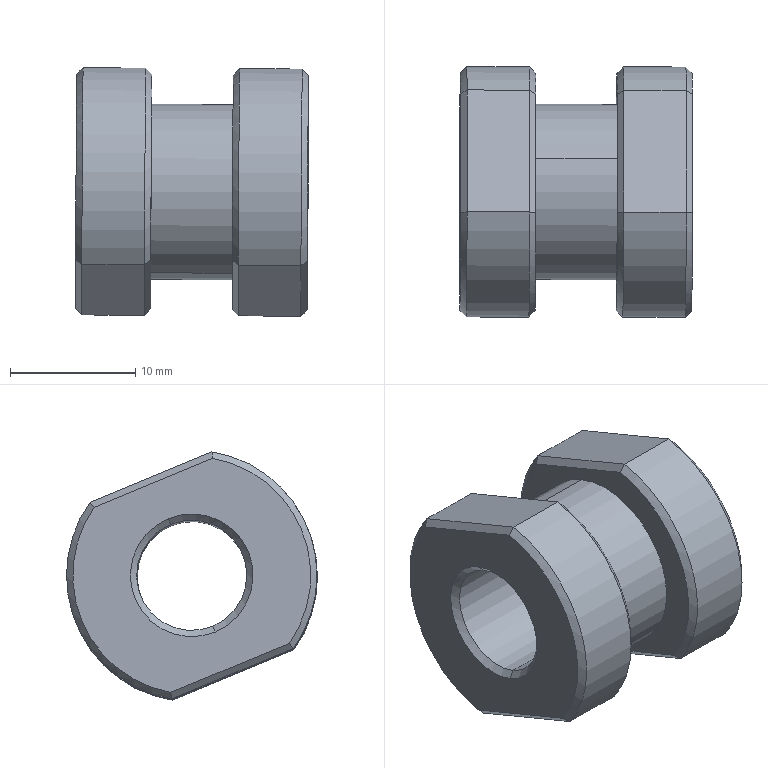Component | SolidWorks | CylinderConnector-1 | 1 solid | 36 faces | box 18.6 x 20.04 x 19.84 mm | volume 3351 mm3 | plane 16 | cone 12 | cylinder 8 | commonest cylinder face diameters 20 x4 8.8 x2 14 x2
build123d program:
from build123d import *

# Parameters (mm, degrees)
SKETCH1_R                   = 7
BOSS_EXTRUDE1_DEPTH         = 6.5
SKETCH2_R                   = 10
BOSS_EXTRUDE2_DEPTH         = 6
CUT_EXTRUDE1_DEPTH          = 24.286
M10X1_25_TAPPED_HOLE1_D     = 8.8
M10X1_25_TAPPED_HOLE1_DEPTH = 23.75
M10X1_25_TAPPED_HOLE1_TIP   = 2.644
CHAMFER1_SIZE               = 0.5


with BuildPart() as part:
    # Sketch1 → Boss-Extrude1 (new body)
    with BuildSketch(Plane.XY):
        with Locations(Location((0, 0, 0), (0, 0, 180))):
            Circle(SKETCH1_R)
    extrude(amount=BOSS_EXTRUDE1_DEPTH)

    # Sketch2 → Boss-Extrude2 (add)
    with BuildSketch(Plane.XY.offset(6.5)):
        Circle(SKETCH2_R)
    boss_extrude2 = extrude(amount=BOSS_EXTRUDE2_DEPTH)

    # Mirror1: Boss-Extrude2 across plane
    add(boss_extrude2.mirror(Plane(origin=(0, 0, 3.25), x_dir=(1, 0, 0), z_dir=(0, 0, -1))))

    # Sketch3 → Cut-Extrude1 (cut, through all)
    with BuildSketch(Plane.XY.offset(12.5)):
        with BuildLine():
            Line((8.5, 5.268), (8.5, -5.268))
            ThreePointArc((8.5, -5.268), (10, 0), (8.5, 5.268))
        make_face()
        with BuildLine():
            Line((-8.5, 5.268), (-8.5, -5.268))
            ThreePointArc((-8.5, -5.268), (-10, 0), (-8.5, 5.268))
        make_face()
    extrude(amount=-CUT_EXTRUDE1_DEPTH, mode=Mode.SUBTRACT)

    # M10x1.25 Tapped Hole1
    with Locations(Plane(origin=(0, 0, -6), x_dir=(-1, 0, 0), z_dir=(0, 0, -1))):
        with Locations((0, 0)):
            Hole(M10X1_25_TAPPED_HOLE1_D / 2, depth=M10X1_25_TAPPED_HOLE1_DEPTH)
            with Locations((0, 0, -(M10X1_25_TAPPED_HOLE1_DEPTH + M10X1_25_TAPPED_HOLE1_TIP / 2))):  # 118° drill point
                Cone(0, M10X1_25_TAPPED_HOLE1_D / 2, M10X1_25_TAPPED_HOLE1_TIP, mode=Mode.SUBTRACT)

    # Chamfer1
    chamfer1_edges = [part.edges().sort_by_distance(p)[0] for p in [
        (0, -10, -6),
        (0, -10, 0),
        (0, -10, 12.5),
        (0, -10, 6.5),
        (-8.5, 0, 6.5),
        (-8.5, 0, 0),
        (-8.5, 0, -6),
        (-8.5, 0, 12.5),
        (0, 10, -6),
        (0, 10, 0),
        (0, 10, 12.5),
        (0, 10, 6.5),
        (8.5, 0, 6.5),
        (8.5, 0, 0),
        (8.5, 0, -6),
        (8.5, 0, 12.5),
        (-4.4, 0, 12.5),
        (-4.4, 0, -6),
    ]]
    chamfer(chamfer1_edges, length=CHAMFER1_SIZE)


solid = part.part

# Placed as in the assembly
solid = solid.moved(Location((53.949, -72.168, 459.571), (158.758, 89.634, 178.758)))
STEP:
#1=CARTESIAN_POINT('',(2.595,-2.909,17.93));
#2=VERTEX_POINT('',#1);
#3=CARTESIAN_POINT('',(2.598,-2.776,18.251));
#4=VERTEX_POINT('',#3);
#5=CARTESIAN_POINT('',(2.596,-2.842,18.091));
#6=DIRECTION('',(1.,-0.002314,-0.005953));
#7=DIRECTION('',(0.006385,0.3824,0.924));
#8=AXIS2_PLACEMENT_3D('',#5,#6,#7);
#9=CIRCLE('',#8,0.1732);
#10=EDGE_CURVE('',#2,#4,#9,.T.);
#11=ORIENTED_EDGE('',*,*,#10,.F.);
#12=CARTESIAN_POINT('',(2.615,-2.916,17.912));
#13=VERTEX_POINT('',#12);
#14=CARTESIAN_POINT('',(2.595,-2.909,17.93));
#15=DIRECTION('',(0.7026,-0.272,-0.6576));
#16=VECTOR('',#15,39.37);
#17=LINE('',#14,#16);
#18=EDGE_CURVE('',#2,#13,#17,.T.);
#19=ORIENTED_EDGE('',*,*,#18,.T.);
#20=CARTESIAN_POINT('',(2.617,-2.769,18.269));
#21=VERTEX_POINT('',#20);
#22=CARTESIAN_POINT('',(2.616,-2.842,18.09));
#23=DIRECTION('',(-1.,0.002314,0.005953));
#24=DIRECTION('',(0.006385,0.3824,0.924));
#25=AXIS2_PLACEMENT_3D('',#22,#23,#24);
#26=CIRCLE('',#25,0.1929);
#27=EDGE_CURVE('',#21,#13,#26,.T.);
#28=ORIENTED_EDGE('',*,*,#27,.F.);
#29=CARTESIAN_POINT('',(2.598,-2.776,18.251));
#30=DIRECTION('',(0.7116,0.2688,0.6491));
#31=VECTOR('',#30,39.37);
#32=LINE('',#29,#31);
#33=EDGE_CURVE('',#4,#21,#32,.T.);
#34=ORIENTED_EDGE('',*,*,#33,.F.);
#35=EDGE_LOOP('',(#11,#19,#28,#34));
#36=FACE_OUTER_BOUND('',#35,.T.);
#37=CARTESIAN_POINT('',(2.596,-2.842,18.091));
#38=DIRECTION('',(1.,-0.002314,-0.005953));
#39=DIRECTION('',(0.006385,0.3824,0.924));
#40=AXIS2_PLACEMENT_3D('',#37,#38,#39);
#41=CONICAL_SURFACE('',#40,0.1732,0.7854);
#42=ADVANCED_FACE('',(#36),#41,.F.);
#43=CARTESIAN_POINT('',(1.909,-2.774,18.255));
#44=VERTEX_POINT('',#43);
#45=CARTESIAN_POINT('',(1.906,-2.907,17.935));
#46=VERTEX_POINT('',#45);
#47=CARTESIAN_POINT('',(1.907,-2.841,18.095));
#48=DIRECTION('',(-1.,0.002314,0.005953));
#49=DIRECTION('',(-0.006385,-0.3824,-0.924));
#50=AXIS2_PLACEMENT_3D('',#47,#48,#49);
#51=CIRCLE('',#50,0.1732);
#52=EDGE_CURVE('',#44,#46,#51,.T.);
#53=ORIENTED_EDGE('',*,*,#52,.F.);
#54=CARTESIAN_POINT('',(1.889,-2.767,18.273));
#55=VERTEX_POINT('',#54);
#56=CARTESIAN_POINT('',(1.909,-2.774,18.255));
#57=DIRECTION('',(-0.7026,0.272,0.6576));
#58=VECTOR('',#57,39.37);
#59=LINE('',#56,#58);
#60=EDGE_CURVE('',#44,#55,#59,.T.);
#61=ORIENTED_EDGE('',*,*,#60,.T.);
#62=CARTESIAN_POINT('',(1.887,-2.914,17.916));
#63=VERTEX_POINT('',#62);
#64=CARTESIAN_POINT('',(1.888,-2.841,18.095));
#65=DIRECTION('',(1.,-0.002314,-0.005953));
#66=DIRECTION('',(-0.006385,-0.3824,-0.924));
#67=AXIS2_PLACEMENT_3D('',#64,#65,#66);
#68=CIRCLE('',#67,0.1929);
#69=EDGE_CURVE('',#63,#55,#68,.T.);
#70=ORIENTED_EDGE('',*,*,#69,.F.);
#71=CARTESIAN_POINT('',(1.906,-2.907,17.935));
#72=DIRECTION('',(-0.7116,-0.2688,-0.6491));
#73=VECTOR('',#72,39.37);
#74=LINE('',#71,#73);
#75=EDGE_CURVE('',#46,#63,#74,.T.);
#76=ORIENTED_EDGE('',*,*,#75,.F.);
#77=EDGE_LOOP('',(#53,#61,#70,#76));
#78=FACE_OUTER_BOUND('',#77,.T.);
#79=CARTESIAN_POINT('',(1.907,-2.841,18.095));
#80=DIRECTION('',(-1.,0.002314,0.005953));
#81=DIRECTION('',(-0.006385,-0.3824,-0.924));
#82=AXIS2_PLACEMENT_3D('',#79,#80,#81);
#83=CONICAL_SURFACE('',#82,0.1732,0.7854);
#84=ADVANCED_FACE('',(#78),#83,.F.);
#85=ORIENTED_EDGE('',*,*,#10,.T.);
#86=CARTESIAN_POINT('',(1.889,-2.774,18.255));
#87=DIRECTION('',(-1.,0.002314,0.005953));
#88=VECTOR('',#87,39.37);
#89=LINE('',#86,#88);
#90=EDGE_CURVE('',#4,#44,#89,.T.);
#91=ORIENTED_EDGE('',*,*,#90,.T.);
#92=ORIENTED_EDGE('',*,*,#52,.T.);
#93=CARTESIAN_POINT('',(1.887,-2.907,17.935));
#94=DIRECTION('',(-1.,0.002314,0.005953));
#95=VECTOR('',#94,39.37);
#96=LINE('',#93,#95);
#97=EDGE_CURVE('',#2,#46,#96,.T.);
#98=ORIENTED_EDGE('',*,*,#97,.F.);
#99=EDGE_LOOP('',(#85,#91,#92,#98));
#100=FACE_OUTER_BOUND('',#99,.T.);
#101=CARTESIAN_POINT('',(1.888,-2.841,18.095));
#102=DIRECTION('',(-1.,0.002314,0.005953));
#103=DIRECTION('',(-0.006385,-0.3824,-0.924));
#104=AXIS2_PLACEMENT_3D('',#101,#102,#103);
#105=CYLINDRICAL_SURFACE('',#104,0.1732);
#106=ADVANCED_FACE('',(#100),#105,.F.);
#107=CARTESIAN_POINT('',(2.382,-2.736,18.346));
#108=VERTEX_POINT('',#107);
#109=CARTESIAN_POINT('',(2.378,-2.947,17.837));
#110=VERTEX_POINT('',#109);
#111=CARTESIAN_POINT('',(2.38,-2.842,18.092));
#112=DIRECTION('',(1.,-0.002314,-0.005953));
#113=DIRECTION('',(0.006385,0.3824,0.924));
#114=AXIS2_PLACEMENT_3D('',#111,#112,#113);
#115=CIRCLE('',#114,0.2756);
#116=EDGE_CURVE('',#108,#110,#115,.T.);
#117=ORIENTED_EDGE('',*,*,#116,.F.);
#118=CARTESIAN_POINT('',(2.126,-2.736,18.348));
#119=VERTEX_POINT('',#118);
#120=CARTESIAN_POINT('',(2.382,-2.736,18.346));
#121=DIRECTION('',(-1.,0.002314,0.005953));
#122=VECTOR('',#121,39.37);
#123=LINE('',#120,#122);
#124=EDGE_CURVE('',#108,#119,#123,.T.);
#125=ORIENTED_EDGE('',*,*,#124,.T.);
#126=CARTESIAN_POINT('',(2.122,-2.947,17.839));
#127=VERTEX_POINT('',#126);
#128=CARTESIAN_POINT('',(2.124,-2.841,18.093));
#129=DIRECTION('',(-1.,0.002314,0.005953));
#130=DIRECTION('',(-0.006385,-0.3824,-0.924));
#131=AXIS2_PLACEMENT_3D('',#128,#129,#130);
#132=CIRCLE('',#131,0.2756);
#133=EDGE_CURVE('',#127,#119,#132,.T.);
#134=ORIENTED_EDGE('',*,*,#133,.F.);
#135=CARTESIAN_POINT('',(2.378,-2.947,17.837));
#136=DIRECTION('',(-1.,0.002314,0.005953));
#137=VECTOR('',#136,39.37);
#138=LINE('',#135,#137);
#139=EDGE_CURVE('',#110,#127,#138,.T.);
#140=ORIENTED_EDGE('',*,*,#139,.F.);
#141=EDGE_LOOP('',(#117,#125,#134,#140));
#142=FACE_OUTER_BOUND('',#141,.T.);
#143=CARTESIAN_POINT('',(2.38,-2.842,18.092));
#144=DIRECTION('',(-1.,0.002314,0.005953));
#145=DIRECTION('',(-0.006385,-0.3824,-0.924));
#146=AXIS2_PLACEMENT_3D('',#143,#144,#145);
#147=CYLINDRICAL_SURFACE('',#146,0.2756);
#148=ADVANCED_FACE('',(#142),#147,.T.);
#149=CARTESIAN_POINT('',(2.397,-3.161,17.862));
#150=VERTEX_POINT('',#149);
#151=CARTESIAN_POINT('',(2.594,-3.162,17.861));
#152=VERTEX_POINT('',#151);
#153=CARTESIAN_POINT('',(1.886,-3.16,17.865));
#154=DIRECTION('',(1.,-0.002314,-0.005953));
#155=VECTOR('',#154,39.37);
#156=LINE('',#153,#155);
#157=EDGE_CURVE('',#150,#152,#156,.T.);
#158=ORIENTED_EDGE('',*,*,#157,.T.);
#159=CARTESIAN_POINT('',(2.599,-2.906,18.479));
#160=VERTEX_POINT('',#159);
#161=CARTESIAN_POINT('',(2.596,-2.842,18.091));
#162=DIRECTION('',(-1.,0.002314,0.005953));
#163=DIRECTION('',(0.006385,0.3824,0.924));
#164=AXIS2_PLACEMENT_3D('',#161,#162,#163);
#165=CIRCLE('',#164,0.3937);
#166=EDGE_CURVE('',#152,#160,#165,.T.);
#167=ORIENTED_EDGE('',*,*,#166,.T.);
#168=CARTESIAN_POINT('',(2.402,-2.906,18.48));
#169=VERTEX_POINT('',#168);
#170=CARTESIAN_POINT('',(1.89,-2.904,18.483));
#171=DIRECTION('',(1.,-0.002314,-0.005953));
#172=VECTOR('',#171,39.37);
#173=LINE('',#170,#172);
#174=EDGE_CURVE('',#169,#160,#173,.T.);
#175=ORIENTED_EDGE('',*,*,#174,.F.);
#176=CARTESIAN_POINT('',(2.4,-2.842,18.092));
#177=DIRECTION('',(1.,-0.002314,-0.005953));
#178=DIRECTION('',(0.006385,0.3824,0.924));
#179=AXIS2_PLACEMENT_3D('',#176,#177,#178);
#180=CIRCLE('',#179,0.3937);
#181=EDGE_CURVE('',#169,#150,#180,.T.);
#182=ORIENTED_EDGE('',*,*,#181,.T.);
#183=EDGE_LOOP('',(#158,#167,#175,#182));
#184=FACE_OUTER_BOUND('',#183,.T.);
#185=CARTESIAN_POINT('',(2.616,-2.842,18.09));
#186=DIRECTION('',(-1.,0.002314,0.005953));
#187=DIRECTION('',(-0.006385,-0.3824,-0.924));
#188=AXIS2_PLACEMENT_3D('',#185,#186,#187);
#189=CYLINDRICAL_SURFACE('',#188,0.3937);
#190=ADVANCED_FACE('',(#184),#189,.T.);
#191=CARTESIAN_POINT('',(1.905,-2.777,17.706));
#192=VERTEX_POINT('',#191);
#193=CARTESIAN_POINT('',(2.102,-2.778,17.705));
#194=VERTEX_POINT('',#193);
#195=CARTESIAN_POINT('',(1.886,-2.777,17.706));
#196=DIRECTION('',(1.,-0.002314,-0.005953));
#197=VECTOR('',#196,39.37);
#198=LINE('',#195,#197);
#199=EDGE_CURVE('',#192,#194,#198,.T.);
#200=ORIENTED_EDGE('',*,*,#199,.F.);
#201=CARTESIAN_POINT('',(1.91,-2.521,18.325));
#202=VERTEX_POINT('',#201);
#203=CARTESIAN_POINT('',(1.907,-2.841,18.095));
#204=DIRECTION('',(1.,-0.002314,-0.005953));
#205=DIRECTION('',(-0.006385,-0.3824,-0.924));
#206=AXIS2_PLACEMENT_3D('',#203,#204,#205);
#207=CIRCLE('',#206,0.3937);
#208=EDGE_CURVE('',#192,#202,#207,.T.);
#209=ORIENTED_EDGE('',*,*,#208,.T.);
#210=CARTESIAN_POINT('',(2.106,-2.522,18.323));
#211=VERTEX_POINT('',#210);
#212=CARTESIAN_POINT('',(1.89,-2.521,18.325));
#213=DIRECTION('',(1.,-0.002314,-0.005953));
#214=VECTOR('',#213,39.37);
#215=LINE('',#212,#214);
#216=EDGE_CURVE('',#202,#211,#215,.T.);
#217=ORIENTED_EDGE('',*,*,#216,.T.);
#218=CARTESIAN_POINT('',(2.104,-2.841,18.093));
#219=DIRECTION('',(-1.,0.002314,0.005953));
#220=DIRECTION('',(-0.006385,-0.3824,-0.924));
#221=AXIS2_PLACEMENT_3D('',#218,#219,#220);
#222=CIRCLE('',#221,0.3937);
#223=EDGE_CURVE('',#211,#194,#222,.T.);
#224=ORIENTED_EDGE('',*,*,#223,.T.);
#225=EDGE_LOOP('',(#200,#209,#217,#224));
#226=FACE_OUTER_BOUND('',#225,.T.);
#227=CARTESIAN_POINT('',(1.888,-2.841,18.095));
#228=DIRECTION('',(1.,-0.002314,-0.005953));
#229=DIRECTION('',(0.006385,0.3824,0.924));
#230=AXIS2_PLACEMENT_3D('',#227,#228,#229);
#231=CYLINDRICAL_SURFACE('',#230,0.3937);
#232=ADVANCED_FACE('',(#226),#231,.T.);
#233=ORIENTED_EDGE('',*,*,#124,.F.);
#234=CARTESIAN_POINT('',(2.38,-2.842,18.092));
#235=DIRECTION('',(1.,-0.002314,-0.005953));
#236=DIRECTION('',(0.006385,0.3824,0.924));
#237=AXIS2_PLACEMENT_3D('',#234,#235,#236);
#238=CIRCLE('',#237,0.2756);
#239=EDGE_CURVE('',#110,#108,#238,.T.);
#240=ORIENTED_EDGE('',*,*,#239,.F.);
#241=ORIENTED_EDGE('',*,*,#139,.T.);
#242=CARTESIAN_POINT('',(2.124,-2.841,18.093));
#243=DIRECTION('',(-1.,0.002314,0.005953));
#244=DIRECTION('',(-0.006385,-0.3824,-0.924));
#245=AXIS2_PLACEMENT_3D('',#242,#243,#244);
#246=CIRCLE('',#245,0.2756);
#247=EDGE_CURVE('',#119,#127,#246,.T.);
#248=ORIENTED_EDGE('',*,*,#247,.F.);
#249=EDGE_LOOP('',(#233,#240,#241,#248));
#250=FACE_OUTER_BOUND('',#249,.T.);
#251=CARTESIAN_POINT('',(2.38,-2.842,18.092));
#252=DIRECTION('',(-1.,0.002314,0.005953));
#253=DIRECTION('',(-0.006385,-0.3824,-0.924));
#254=AXIS2_PLACEMENT_3D('',#251,#252,#253);
#255=CYLINDRICAL_SURFACE('',#254,0.2756);
#256=ADVANCED_FACE('',(#250),#255,.T.);
#257=CARTESIAN_POINT('',(2.382,-2.535,18.306));
#258=VERTEX_POINT('',#257);
#259=CARTESIAN_POINT('',(2.378,-2.776,17.724));
#260=VERTEX_POINT('',#259);
#261=CARTESIAN_POINT('',(2.38,-2.842,18.092));
#262=DIRECTION('',(-1.,0.002314,0.005953));
#263=DIRECTION('',(0.006385,0.3824,0.924));
#264=AXIS2_PLACEMENT_3D('',#261,#262,#263);
#265=CIRCLE('',#264,0.374);
#266=EDGE_CURVE('',#258,#260,#265,.T.);
#267=ORIENTED_EDGE('',*,*,#266,.T.);
#268=CARTESIAN_POINT('',(2.378,-3.149,17.878));
#269=VERTEX_POINT('',#268);
#270=CARTESIAN_POINT('',(2.378,-2.962,17.801));
#271=DIRECTION('',(0.0001384,-0.924,0.3824));
#272=VECTOR('',#271,39.37);
#273=LINE('',#270,#272);
#274=EDGE_CURVE('',#260,#269,#273,.T.);
#275=ORIENTED_EDGE('',*,*,#274,.T.);
#276=CARTESIAN_POINT('',(2.382,-2.908,18.46));
#277=VERTEX_POINT('',#276);
#278=CARTESIAN_POINT('',(2.38,-2.842,18.092));
#279=DIRECTION('',(-1.,0.002314,0.005953));
#280=DIRECTION('',(0.006385,0.3824,0.924));
#281=AXIS2_PLACEMENT_3D('',#278,#279,#280);
#282=CIRCLE('',#281,0.374);
#283=EDGE_CURVE('',#269,#277,#282,.T.);
#284=ORIENTED_EDGE('',*,*,#283,.T.);
#285=CARTESIAN_POINT('',(2.382,-2.721,18.383));
#286=DIRECTION('',(-0.0001384,0.924,-0.3824));
#287=VECTOR('',#286,39.37);
#288=LINE('',#285,#287);
#289=EDGE_CURVE('',#277,#258,#288,.T.);
#290=ORIENTED_EDGE('',*,*,#289,.T.);
#291=EDGE_LOOP('',(#267,#275,#284,#290));
#292=FACE_OUTER_BOUND('',#291,.T.);
#293=ORIENTED_EDGE('',*,*,#239,.T.);
#294=ORIENTED_EDGE('',*,*,#116,.T.);
#295=EDGE_LOOP('',(#293,#294));
#296=FACE_BOUND('',#295,.T.);
#297=CARTESIAN_POINT('',(2.38,-2.842,18.092));
#298=DIRECTION('',(1.,-0.002314,-0.005953));
#299=DIRECTION('',(0.006385,0.3824,0.924));
#300=AXIS2_PLACEMENT_3D('',#297,#298,#299);
#301=PLANE('',#300);
#302=ADVANCED_FACE('',(#292,#296),#301,.F.);
#303=CARTESIAN_POINT('',(2.402,-2.522,18.322));
#304=VERTEX_POINT('',#303);
#305=CARTESIAN_POINT('',(2.599,-2.523,18.32));
#306=VERTEX_POINT('',#305);
#307=CARTESIAN_POINT('',(1.89,-2.521,18.325));
#308=DIRECTION('',(1.,-0.002314,-0.005953));
#309=VECTOR('',#308,39.37);
#310=LINE('',#307,#309);
#311=EDGE_CURVE('',#304,#306,#310,.T.);
#312=ORIENTED_EDGE('',*,*,#311,.T.);
#313=CARTESIAN_POINT('',(2.594,-2.779,17.702));
#314=VERTEX_POINT('',#313);
#315=CARTESIAN_POINT('',(2.596,-2.842,18.091));
#316=DIRECTION('',(-1.,0.002314,0.005953));
#317=DIRECTION('',(0.006385,0.3824,0.924));
#318=AXIS2_PLACEMENT_3D('',#315,#316,#317);
#319=CIRCLE('',#318,0.3937);
#320=EDGE_CURVE('',#306,#314,#319,.T.);
#321=ORIENTED_EDGE('',*,*,#320,.T.);
#322=CARTESIAN_POINT('',(2.397,-2.778,17.703));
#323=VERTEX_POINT('',#322);
#324=CARTESIAN_POINT('',(1.886,-2.777,17.706));
#325=DIRECTION('',(1.,-0.002314,-0.005953));
#326=VECTOR('',#325,39.37);
#327=LINE('',#324,#326);
#328=EDGE_CURVE('',#323,#314,#327,.T.);
#329=ORIENTED_EDGE('',*,*,#328,.F.);
#330=CARTESIAN_POINT('',(2.4,-2.842,18.092));
#331=DIRECTION('',(1.,-0.002314,-0.005953));
#332=DIRECTION('',(0.006385,0.3824,0.924));
#333=AXIS2_PLACEMENT_3D('',#330,#331,#332);
#334=CIRCLE('',#333,0.3937);
#335=EDGE_CURVE('',#323,#304,#334,.T.);
#336=ORIENTED_EDGE('',*,*,#335,.T.);
#337=EDGE_LOOP('',(#312,#321,#329,#336));
#338=FACE_OUTER_BOUND('',#337,.T.);
#339=CARTESIAN_POINT('',(2.616,-2.842,18.09));
#340=DIRECTION('',(-1.,0.002314,0.005953));
#341=DIRECTION('',(-0.006385,-0.3824,-0.924));
#342=AXIS2_PLACEMENT_3D('',#339,#340,#341);
#343=CYLINDRICAL_SURFACE('',#342,0.3937);
#344=ADVANCED_FACE('',(#338),#343,.T.);
#345=CARTESIAN_POINT('',(2.614,-3.149,17.877));
#346=VERTEX_POINT('',#345);
#347=CARTESIAN_POINT('',(2.614,-2.776,17.722));
#348=VERTEX_POINT('',#347);
#349=CARTESIAN_POINT('',(2.614,-2.771,17.72));
#350=DIRECTION('',(-0.0001384,0.924,-0.3824));
#351=VECTOR('',#350,39.37);
#352=LINE('',#349,#351);
#353=EDGE_CURVE('',#346,#348,#352,.T.);
#354=ORIENTED_EDGE('',*,*,#353,.T.);
#355=CARTESIAN_POINT('',(2.618,-2.536,18.304));
#356=VERTEX_POINT('',#355);
#357=CARTESIAN_POINT('',(2.616,-2.842,18.09));
#358=DIRECTION('',(1.,-0.002314,-0.005953));
#359=DIRECTION('',(0.006385,0.3824,0.924));
#360=AXIS2_PLACEMENT_3D('',#357,#358,#359);
#361=CIRCLE('',#360,0.374);
#362=EDGE_CURVE('',#348,#356,#361,.T.);
#363=ORIENTED_EDGE('',*,*,#362,.T.);
#364=CARTESIAN_POINT('',(2.618,-2.908,18.459));
#365=VERTEX_POINT('',#364);
#366=CARTESIAN_POINT('',(2.618,-2.914,18.461));
#367=DIRECTION('',(0.0001384,-0.924,0.3824));
#368=VECTOR('',#367,39.37);
#369=LINE('',#366,#368);
#370=EDGE_CURVE('',#356,#365,#369,.T.);
#371=ORIENTED_EDGE('',*,*,#370,.T.);
#372=CARTESIAN_POINT('',(2.616,-2.842,18.09));
#373=DIRECTION('',(1.,-0.002314,-0.005953));
#374=DIRECTION('',(0.006385,0.3824,0.924));
#375=AXIS2_PLACEMENT_3D('',#372,#373,#374);
#376=CIRCLE('',#375,0.374);
#377=EDGE_CURVE('',#365,#346,#376,.T.);
#378=ORIENTED_EDGE('',*,*,#377,.T.);
#379=EDGE_LOOP('',(#354,#363,#371,#378));
#380=FACE_OUTER_BOUND('',#379,.T.);
#381=ORIENTED_EDGE('',*,*,#27,.T.);
#382=CARTESIAN_POINT('',(2.616,-2.842,18.09));
#383=DIRECTION('',(-1.,0.002314,0.005953));
#384=DIRECTION('',(0.006385,0.3824,0.924));
#385=AXIS2_PLACEMENT_3D('',#382,#383,#384);
#386=CIRCLE('',#385,0.1929);
#387=EDGE_CURVE('',#13,#21,#386,.T.);
#388=ORIENTED_EDGE('',*,*,#387,.T.);
#389=EDGE_LOOP('',(#381,#388));
#390=FACE_BOUND('',#389,.T.);
#391=CARTESIAN_POINT('',(2.616,-2.842,18.09));
#392=DIRECTION('',(1.,-0.002314,-0.005953));
#393=DIRECTION('',(0.006385,0.3824,0.924));
#394=AXIS2_PLACEMENT_3D('',#391,#392,#393);
#395=PLANE('',#394);
#396=ADVANCED_FACE('',(#380,#390),#395,.T.);
#397=CARTESIAN_POINT('',(2.126,-2.907,18.461));
#398=VERTEX_POINT('',#397);
#399=CARTESIAN_POINT('',(2.122,-3.148,17.879));
#400=VERTEX_POINT('',#399);
#401=CARTESIAN_POINT('',(2.124,-2.841,18.093));
#402=DIRECTION('',(1.,-0.002314,-0.005953));
#403=DIRECTION('',(-0.006385,-0.3824,-0.924));
#404=AXIS2_PLACEMENT_3D('',#401,#402,#403);
#405=CIRCLE('',#404,0.374);
#406=EDGE_CURVE('',#398,#400,#405,.T.);
#407=ORIENTED_EDGE('',*,*,#406,.T.);
#408=CARTESIAN_POINT('',(2.122,-2.775,17.725));
#409=VERTEX_POINT('',#408);
#410=CARTESIAN_POINT('',(2.122,-2.962,17.802));
#411=DIRECTION('',(-0.0001384,0.924,-0.3824));
#412=VECTOR('',#411,39.37);
#413=LINE('',#410,#412);
#414=EDGE_CURVE('',#400,#409,#413,.T.);
#415=ORIENTED_EDGE('',*,*,#414,.T.);
#416=CARTESIAN_POINT('',(2.126,-2.534,18.307));
#417=VERTEX_POINT('',#416);
#418=CARTESIAN_POINT('',(2.124,-2.841,18.093));
#419=DIRECTION('',(1.,-0.002314,-0.005953));
#420=DIRECTION('',(-0.006385,-0.3824,-0.924));
#421=AXIS2_PLACEMENT_3D('',#418,#419,#420);
#422=CIRCLE('',#421,0.374);
#423=EDGE_CURVE('',#409,#417,#422,.T.);
#424=ORIENTED_EDGE('',*,*,#423,.T.);
#425=CARTESIAN_POINT('',(2.126,-2.721,18.384));
#426=DIRECTION('',(0.0001384,-0.924,0.3824));
#427=VECTOR('',#426,39.37);
#428=LINE('',#425,#427);
#429=EDGE_CURVE('',#417,#398,#428,.T.);
#430=ORIENTED_EDGE('',*,*,#429,.T.);
#431=EDGE_LOOP('',(#407,#415,#424,#430));
#432=FACE_OUTER_BOUND('',#431,.T.);
#433=ORIENTED_EDGE('',*,*,#133,.T.);
#434=ORIENTED_EDGE('',*,*,#247,.T.);
#435=EDGE_LOOP('',(#433,#434));
#436=FACE_BOUND('',#435,.T.);
#437=CARTESIAN_POINT('',(2.124,-2.841,18.093));
#438=DIRECTION('',(-1.,0.002314,0.005953));
#439=DIRECTION('',(0.006385,0.3824,0.924));
#440=AXIS2_PLACEMENT_3D('',#437,#438,#439);
#441=PLANE('',#440);
#442=ADVANCED_FACE('',(#432,#436),#441,.F.);
#443=CARTESIAN_POINT('',(1.91,-2.904,18.483));
#444=VERTEX_POINT('',#443);
#445=CARTESIAN_POINT('',(2.106,-2.905,18.482));
#446=VERTEX_POINT('',#445);
#447=CARTESIAN_POINT('',(1.89,-2.904,18.483));
#448=DIRECTION('',(1.,-0.002314,-0.005953));
#449=VECTOR('',#448,39.37);
#450=LINE('',#447,#449);
#451=EDGE_CURVE('',#444,#446,#450,.T.);
#452=ORIENTED_EDGE('',*,*,#451,.F.);
#453=CARTESIAN_POINT('',(1.905,-3.16,17.865));
#454=VERTEX_POINT('',#453);
#455=CARTESIAN_POINT('',(1.907,-2.841,18.095));
#456=DIRECTION('',(1.,-0.002314,-0.005953));
#457=DIRECTION('',(-0.006385,-0.3824,-0.924));
#458=AXIS2_PLACEMENT_3D('',#455,#456,#457);
#459=CIRCLE('',#458,0.3937);
#460=EDGE_CURVE('',#444,#454,#459,.T.);
#461=ORIENTED_EDGE('',*,*,#460,.T.);
#462=CARTESIAN_POINT('',(2.102,-3.161,17.864));
#463=VERTEX_POINT('',#462);
#464=CARTESIAN_POINT('',(1.886,-3.16,17.865));
#465=DIRECTION('',(1.,-0.002314,-0.005953));
#466=VECTOR('',#465,39.37);
#467=LINE('',#464,#466);
#468=EDGE_CURVE('',#454,#463,#467,.T.);
#469=ORIENTED_EDGE('',*,*,#468,.T.);
#470=CARTESIAN_POINT('',(2.104,-2.841,18.093));
#471=DIRECTION('',(-1.,0.002314,0.005953));
#472=DIRECTION('',(-0.006385,-0.3824,-0.924));
#473=AXIS2_PLACEMENT_3D('',#470,#471,#472);
#474=CIRCLE('',#473,0.3937);
#475=EDGE_CURVE('',#463,#446,#474,.T.);
#476=ORIENTED_EDGE('',*,*,#475,.T.);
#477=EDGE_LOOP('',(#452,#461,#469,#476));
#478=FACE_OUTER_BOUND('',#477,.T.);
#479=CARTESIAN_POINT('',(1.888,-2.841,18.095));
#480=DIRECTION('',(1.,-0.002314,-0.005953));
#481=DIRECTION('',(0.006385,0.3824,0.924));
#482=AXIS2_PLACEMENT_3D('',#479,#480,#481);
#483=CYLINDRICAL_SURFACE('',#482,0.3937);
#484=ADVANCED_FACE('',(#478),#483,.T.);
#485=CARTESIAN_POINT('',(1.886,-2.775,17.727));
#486=VERTEX_POINT('',#485);
#487=CARTESIAN_POINT('',(1.886,-3.148,17.881));
#488=VERTEX_POINT('',#487);
#489=CARTESIAN_POINT('',(1.886,-3.153,17.883));
#490=DIRECTION('',(0.0001384,-0.924,0.3824));
#491=VECTOR('',#490,39.37);
#492=LINE('',#489,#491);
#493=EDGE_CURVE('',#486,#488,#492,.T.);
#494=ORIENTED_EDGE('',*,*,#493,.T.);
#495=CARTESIAN_POINT('',(1.89,-2.907,18.463));
#496=VERTEX_POINT('',#495);
#497=CARTESIAN_POINT('',(1.888,-2.841,18.095));
#498=DIRECTION('',(-1.,0.002314,0.005953));
#499=DIRECTION('',(-0.006385,-0.3824,-0.924));
#500=AXIS2_PLACEMENT_3D('',#497,#498,#499);
#501=CIRCLE('',#500,0.374);
#502=EDGE_CURVE('',#488,#496,#501,.T.);
#503=ORIENTED_EDGE('',*,*,#502,.T.);
#504=CARTESIAN_POINT('',(1.89,-2.534,18.309));
#505=VERTEX_POINT('',#504);
#506=CARTESIAN_POINT('',(1.89,-2.529,18.306));
#507=DIRECTION('',(-0.0001384,0.924,-0.3824));
#508=VECTOR('',#507,39.37);
#509=LINE('',#506,#508);
#510=EDGE_CURVE('',#496,#505,#509,.T.);
#511=ORIENTED_EDGE('',*,*,#510,.T.);
#512=CARTESIAN_POINT('',(1.888,-2.841,18.095));
#513=DIRECTION('',(-1.,0.002314,0.005953));
#514=DIRECTION('',(-0.006385,-0.3824,-0.924));
#515=AXIS2_PLACEMENT_3D('',#512,#513,#514);
#516=CIRCLE('',#515,0.374);
#517=EDGE_CURVE('',#505,#486,#516,.T.);
#518=ORIENTED_EDGE('',*,*,#517,.T.);
#519=EDGE_LOOP('',(#494,#503,#511,#518));
#520=FACE_OUTER_BOUND('',#519,.T.);
#521=ORIENTED_EDGE('',*,*,#69,.T.);
#522=CARTESIAN_POINT('',(1.888,-2.841,18.095));
#523=DIRECTION('',(1.,-0.002314,-0.005953));
#524=DIRECTION('',(-0.006385,-0.3824,-0.924));
#525=AXIS2_PLACEMENT_3D('',#522,#523,#524);
#526=CIRCLE('',#525,0.1929);
#527=EDGE_CURVE('',#55,#63,#526,.T.);
#528=ORIENTED_EDGE('',*,*,#527,.T.);
#529=EDGE_LOOP('',(#521,#528));
#530=FACE_BOUND('',#529,.T.);
#531=CARTESIAN_POINT('',(1.888,-2.841,18.095));
#532=DIRECTION('',(-1.,0.002314,0.005953));
#533=DIRECTION('',(0.006385,0.3824,0.924));
#534=AXIS2_PLACEMENT_3D('',#531,#532,#533);
#535=PLANE('',#534);
#536=ADVANCED_FACE('',(#520,#530),#535,.T.);
#537=ORIENTED_EDGE('',*,*,#468,.F.);
#538=CARTESIAN_POINT('',(1.905,-2.777,17.706));
#539=DIRECTION('',(-0.0001384,0.924,-0.3824));
#540=VECTOR('',#539,39.37);
#541=LINE('',#538,#540);
#542=EDGE_CURVE('',#454,#192,#541,.T.);
#543=ORIENTED_EDGE('',*,*,#542,.T.);
#544=ORIENTED_EDGE('',*,*,#199,.T.);
#545=CARTESIAN_POINT('',(2.102,-3.161,17.864));
#546=DIRECTION('',(0.0001384,-0.924,0.3824));
#547=VECTOR('',#546,39.37);
#548=LINE('',#545,#547);
#549=EDGE_CURVE('',#194,#463,#548,.T.);
#550=ORIENTED_EDGE('',*,*,#549,.T.);
#551=EDGE_LOOP('',(#537,#543,#544,#550));
#552=FACE_OUTER_BOUND('',#551,.T.);
#553=CARTESIAN_POINT('',(1.886,-3.16,17.865));
#554=DIRECTION('',(0.006385,0.3824,0.924));
#555=DIRECTION('',(-1.,0.002314,0.005953));
#556=AXIS2_PLACEMENT_3D('',#553,#554,#555);
#557=PLANE('',#556);
#558=ADVANCED_FACE('',(#552),#557,.F.);
#559=ORIENTED_EDGE('',*,*,#328,.T.);
#560=CARTESIAN_POINT('',(2.594,-3.162,17.861));
#561=DIRECTION('',(0.0001384,-0.924,0.3824));
#562=VECTOR('',#561,39.37);
#563=LINE('',#560,#562);
#564=EDGE_CURVE('',#314,#152,#563,.T.);
#565=ORIENTED_EDGE('',*,*,#564,.T.);
#566=ORIENTED_EDGE('',*,*,#157,.F.);
#567=CARTESIAN_POINT('',(2.397,-3.161,17.862));
#568=DIRECTION('',(-0.0001384,0.924,-0.3824));
#569=VECTOR('',#568,39.37);
#570=LINE('',#567,#569);
#571=EDGE_CURVE('',#150,#323,#570,.T.);
#572=ORIENTED_EDGE('',*,*,#571,.T.);
#573=EDGE_LOOP('',(#559,#565,#566,#572));
#574=FACE_OUTER_BOUND('',#573,.T.);
#575=CARTESIAN_POINT('',(1.886,-3.16,17.865));
#576=DIRECTION('',(0.006385,0.3824,0.924));
#577=DIRECTION('',(-1.,0.002314,0.005953));
#578=AXIS2_PLACEMENT_3D('',#575,#576,#577);
#579=PLANE('',#578);
#580=ADVANCED_FACE('',(#574),#579,.F.);
#581=ORIENTED_EDGE('',*,*,#216,.F.);
#582=CARTESIAN_POINT('',(1.91,-2.904,18.483));
#583=DIRECTION('',(0.0001384,-0.924,0.3824));
#584=VECTOR('',#583,39.37);
#585=LINE('',#582,#584);
#586=EDGE_CURVE('',#202,#444,#585,.T.);
#587=ORIENTED_EDGE('',*,*,#586,.T.);
#588=ORIENTED_EDGE('',*,*,#451,.T.);
#589=CARTESIAN_POINT('',(2.106,-2.905,18.482));
#590=DIRECTION('',(-0.0001384,0.924,-0.3824));
#591=VECTOR('',#590,39.37);
#592=LINE('',#589,#591);
#593=EDGE_CURVE('',#446,#211,#592,.T.);
#594=ORIENTED_EDGE('',*,*,#593,.T.);
#595=EDGE_LOOP('',(#581,#587,#588,#594));
#596=FACE_OUTER_BOUND('',#595,.T.);
#597=CARTESIAN_POINT('',(1.89,-2.904,18.483));
#598=DIRECTION('',(-0.006385,-0.3824,-0.924));
#599=DIRECTION('',(-0.0001384,0.924,-0.3824));
#600=AXIS2_PLACEMENT_3D('',#597,#598,#599);
#601=PLANE('',#600);
#602=ADVANCED_FACE('',(#596),#601,.F.);
#603=ORIENTED_EDGE('',*,*,#174,.T.);
#604=CARTESIAN_POINT('',(2.599,-2.523,18.32));
#605=DIRECTION('',(-0.0001384,0.924,-0.3824));
#606=VECTOR('',#605,39.37);
#607=LINE('',#604,#606);
#608=EDGE_CURVE('',#160,#306,#607,.T.);
#609=ORIENTED_EDGE('',*,*,#608,.T.);
#610=ORIENTED_EDGE('',*,*,#311,.F.);
#611=CARTESIAN_POINT('',(2.402,-2.906,18.48));
#612=DIRECTION('',(0.0001384,-0.924,0.3824));
#613=VECTOR('',#612,39.37);
#614=LINE('',#611,#613);
#615=EDGE_CURVE('',#304,#169,#614,.T.);
#616=ORIENTED_EDGE('',*,*,#615,.T.);
#617=EDGE_LOOP('',(#603,#609,#610,#616));
#618=FACE_OUTER_BOUND('',#617,.T.);
#619=CARTESIAN_POINT('',(1.89,-2.904,18.483));
#620=DIRECTION('',(-0.006385,-0.3824,-0.924));
#621=DIRECTION('',(-0.0001384,0.924,-0.3824));
#622=AXIS2_PLACEMENT_3D('',#619,#620,#621);
#623=PLANE('',#622);
#624=ADVANCED_FACE('',(#618),#623,.F.);
#625=ORIENTED_EDGE('',*,*,#90,.F.);
#626=CARTESIAN_POINT('',(2.596,-2.842,18.091));
#627=DIRECTION('',(1.,-0.002314,-0.005953));
#628=DIRECTION('',(0.006385,0.3824,0.924));
#629=AXIS2_PLACEMENT_3D('',#626,#627,#628);
#630=CIRCLE('',#629,0.1732);
#631=EDGE_CURVE('',#4,#2,#630,.T.);
#632=ORIENTED_EDGE('',*,*,#631,.T.);
#633=ORIENTED_EDGE('',*,*,#97,.T.);
#634=CARTESIAN_POINT('',(1.907,-2.841,18.095));
#635=DIRECTION('',(-1.,0.002314,0.005953));
#636=DIRECTION('',(-0.006385,-0.3824,-0.924));
#637=AXIS2_PLACEMENT_3D('',#634,#635,#636);
#638=CIRCLE('',#637,0.1732);
#639=EDGE_CURVE('',#46,#44,#638,.T.);
#640=ORIENTED_EDGE('',*,*,#639,.T.);
#641=EDGE_LOOP('',(#625,#632,#633,#640));
#642=FACE_OUTER_BOUND('',#641,.T.);
#643=CARTESIAN_POINT('',(1.888,-2.841,18.095));
#644=DIRECTION('',(-1.,0.002314,0.005953));
#645=DIRECTION('',(-0.006385,-0.3824,-0.924));
#646=AXIS2_PLACEMENT_3D('',#643,#644,#645);
#647=CYLINDRICAL_SURFACE('',#646,0.1732);
#648=ADVANCED_FACE('',(#642),#647,.F.);
#649=CARTESIAN_POINT('',(1.886,-2.775,17.727));
#650=CARTESIAN_POINT('',(1.892,-2.776,17.72));
#651=CARTESIAN_POINT('',(1.899,-2.776,17.713));
#652=CARTESIAN_POINT('',(1.905,-2.777,17.706));
#653=B_SPLINE_CURVE_WITH_KNOTS('',3,(#649,#650,#651,#652),.UNSPECIFIED.,.F.,.F.,(4,4),(0.,0.0007217),.UNSPECIFIED.);
#654=EDGE_CURVE('',#486,#192,#653,.T.);
#655=ORIENTED_EDGE('',*,*,#654,.F.);
#656=ORIENTED_EDGE('',*,*,#517,.F.);
#657=CARTESIAN_POINT('',(1.91,-2.521,18.325));
#658=CARTESIAN_POINT('',(1.903,-2.525,18.319));
#659=CARTESIAN_POINT('',(1.896,-2.53,18.314));
#660=CARTESIAN_POINT('',(1.89,-2.534,18.309));
#661=B_SPLINE_CURVE_WITH_KNOTS('',3,(#657,#658,#659,#660),.UNSPECIFIED.,.F.,.F.,(4,4),(0.,0.0007217),.UNSPECIFIED.);
#662=EDGE_CURVE('',#202,#505,#661,.T.);
#663=ORIENTED_EDGE('',*,*,#662,.F.);
#664=ORIENTED_EDGE('',*,*,#208,.F.);
#665=EDGE_LOOP('',(#655,#656,#663,#664));
#666=FACE_OUTER_BOUND('',#665,.T.);
#667=CARTESIAN_POINT('',(1.907,-2.841,18.095));
#668=DIRECTION('',(1.,-0.002314,-0.005953));
#669=DIRECTION('',(0.006385,0.3824,0.924));
#670=AXIS2_PLACEMENT_3D('',#667,#668,#669);
#671=CONICAL_SURFACE('',#670,0.3937,0.7854);
#672=ADVANCED_FACE('',(#666),#671,.T.);
#673=ORIENTED_EDGE('',*,*,#662,.T.);
#674=ORIENTED_EDGE('',*,*,#510,.F.);
#675=CARTESIAN_POINT('',(1.91,-2.904,18.483));
#676=CARTESIAN_POINT('',(1.903,-2.905,18.476));
#677=CARTESIAN_POINT('',(1.896,-2.906,18.47));
#678=CARTESIAN_POINT('',(1.89,-2.907,18.463));
#679=B_SPLINE_CURVE_WITH_KNOTS('',3,(#675,#676,#677,#678),.UNSPECIFIED.,.F.,.F.,(4,4),(0.,0.0007217),.UNSPECIFIED.);
#680=EDGE_CURVE('',#444,#496,#679,.T.);
#681=ORIENTED_EDGE('',*,*,#680,.F.);
#682=ORIENTED_EDGE('',*,*,#586,.F.);
#683=EDGE_LOOP('',(#673,#674,#681,#682));
#684=FACE_OUTER_BOUND('',#683,.T.);
#685=CARTESIAN_POINT('',(1.89,-2.72,18.386));
#686=DIRECTION('',(-0.7026,0.272,0.6576));
#687=DIRECTION('',(0.0001384,-0.924,0.3824));
#688=AXIS2_PLACEMENT_3D('',#685,#686,#687);
#689=PLANE('',#688);
#690=ADVANCED_FACE('',(#684),#689,.T.);
#691=ORIENTED_EDGE('',*,*,#654,.T.);
#692=ORIENTED_EDGE('',*,*,#542,.F.);
#693=CARTESIAN_POINT('',(1.886,-3.148,17.881));
#694=CARTESIAN_POINT('',(1.892,-3.152,17.876));
#695=CARTESIAN_POINT('',(1.899,-3.156,17.87));
#696=CARTESIAN_POINT('',(1.905,-3.16,17.865));
#697=B_SPLINE_CURVE_WITH_KNOTS('',3,(#693,#694,#695,#696),.UNSPECIFIED.,.F.,.F.,(4,4),(0.,0.0007217),.UNSPECIFIED.);
#698=EDGE_CURVE('',#488,#454,#697,.T.);
#699=ORIENTED_EDGE('',*,*,#698,.F.);
#700=ORIENTED_EDGE('',*,*,#493,.F.);
#701=EDGE_LOOP('',(#691,#692,#699,#700));
#702=FACE_OUTER_BOUND('',#701,.T.);
#703=CARTESIAN_POINT('',(1.886,-2.961,17.804));
#704=DIRECTION('',(-0.7116,-0.2688,-0.6491));
#705=DIRECTION('',(-0.0001384,0.924,-0.3824));
#706=AXIS2_PLACEMENT_3D('',#703,#704,#705);
#707=PLANE('',#706);
#708=ADVANCED_FACE('',(#702),#707,.T.);
#709=ORIENTED_EDGE('',*,*,#680,.T.);
#710=ORIENTED_EDGE('',*,*,#502,.F.);
#711=ORIENTED_EDGE('',*,*,#698,.T.);
#712=ORIENTED_EDGE('',*,*,#460,.F.);
#713=EDGE_LOOP('',(#709,#710,#711,#712));
#714=FACE_OUTER_BOUND('',#713,.T.);
#715=CARTESIAN_POINT('',(1.907,-2.841,18.095));
#716=DIRECTION('',(1.,-0.002314,-0.005953));
#717=DIRECTION('',(0.006385,0.3824,0.924));
#718=AXIS2_PLACEMENT_3D('',#715,#716,#717);
#719=CONICAL_SURFACE('',#718,0.3937,0.7854);
#720=ADVANCED_FACE('',(#714),#719,.T.);
#721=ORIENTED_EDGE('',*,*,#60,.F.);
#722=ORIENTED_EDGE('',*,*,#639,.F.);
#723=ORIENTED_EDGE('',*,*,#75,.T.);
#724=ORIENTED_EDGE('',*,*,#527,.F.);
#725=EDGE_LOOP('',(#721,#722,#723,#724));
#726=FACE_OUTER_BOUND('',#725,.T.);
#727=CARTESIAN_POINT('',(1.907,-2.841,18.095));
#728=DIRECTION('',(-1.,0.002314,0.005953));
#729=DIRECTION('',(-0.006385,-0.3824,-0.924));
#730=AXIS2_PLACEMENT_3D('',#727,#728,#729);
#731=CONICAL_SURFACE('',#730,0.1732,0.7854);
#732=ADVANCED_FACE('',(#726),#731,.F.);
#733=CARTESIAN_POINT('',(2.599,-2.906,18.479));
#734=CARTESIAN_POINT('',(2.605,-2.907,18.472));
#735=CARTESIAN_POINT('',(2.612,-2.908,18.465));
#736=CARTESIAN_POINT('',(2.618,-2.908,18.459));
#737=B_SPLINE_CURVE_WITH_KNOTS('',3,(#733,#734,#735,#736),.UNSPECIFIED.,.F.,.F.,(4,4),(0.,0.0007217),.UNSPECIFIED.);
#738=EDGE_CURVE('',#160,#365,#737,.T.);
#739=ORIENTED_EDGE('',*,*,#738,.F.);
#740=ORIENTED_EDGE('',*,*,#166,.F.);
#741=CARTESIAN_POINT('',(2.614,-3.149,17.877));
#742=CARTESIAN_POINT('',(2.608,-3.153,17.871));
#743=CARTESIAN_POINT('',(2.601,-3.158,17.866));
#744=CARTESIAN_POINT('',(2.594,-3.162,17.861));
#745=B_SPLINE_CURVE_WITH_KNOTS('',3,(#741,#742,#743,#744),.UNSPECIFIED.,.F.,.F.,(4,4),(0.,0.0007217),.UNSPECIFIED.);
#746=EDGE_CURVE('',#346,#152,#745,.T.);
#747=ORIENTED_EDGE('',*,*,#746,.F.);
#748=ORIENTED_EDGE('',*,*,#377,.F.);
#749=EDGE_LOOP('',(#739,#740,#747,#748));
#750=FACE_OUTER_BOUND('',#749,.T.);
#751=CARTESIAN_POINT('',(2.616,-2.842,18.09));
#752=DIRECTION('',(-1.,0.002314,0.005953));
#753=DIRECTION('',(-0.006385,-0.3824,-0.924));
#754=AXIS2_PLACEMENT_3D('',#751,#752,#753);
#755=CONICAL_SURFACE('',#754,0.374,0.7854);
#756=ADVANCED_FACE('',(#750),#755,.T.);
#757=ORIENTED_EDGE('',*,*,#746,.T.);
#758=ORIENTED_EDGE('',*,*,#564,.F.);
#759=CARTESIAN_POINT('',(2.614,-2.776,17.722));
#760=CARTESIAN_POINT('',(2.607,-2.777,17.716));
#761=CARTESIAN_POINT('',(2.601,-2.778,17.709));
#762=CARTESIAN_POINT('',(2.594,-2.779,17.702));
#763=B_SPLINE_CURVE_WITH_KNOTS('',3,(#759,#760,#761,#762),.UNSPECIFIED.,.F.,.F.,(4,4),(0.,0.0007217),.UNSPECIFIED.);
#764=EDGE_CURVE('',#348,#314,#763,.T.);
#765=ORIENTED_EDGE('',*,*,#764,.F.);
#766=ORIENTED_EDGE('',*,*,#353,.F.);
#767=EDGE_LOOP('',(#757,#758,#765,#766));
#768=FACE_OUTER_BOUND('',#767,.T.);
#769=CARTESIAN_POINT('',(2.594,-3.162,17.861));
#770=DIRECTION('',(0.7026,-0.272,-0.6576));
#771=DIRECTION('',(-0.0001384,0.924,-0.3824));
#772=AXIS2_PLACEMENT_3D('',#769,#770,#771);
#773=PLANE('',#772);
#774=ADVANCED_FACE('',(#768),#773,.T.);
#775=ORIENTED_EDGE('',*,*,#738,.T.);
#776=ORIENTED_EDGE('',*,*,#370,.F.);
#777=CARTESIAN_POINT('',(2.599,-2.523,18.32));
#778=CARTESIAN_POINT('',(2.605,-2.527,18.315));
#779=CARTESIAN_POINT('',(2.612,-2.531,18.31));
#780=CARTESIAN_POINT('',(2.618,-2.536,18.304));
#781=B_SPLINE_CURVE_WITH_KNOTS('',3,(#777,#778,#779,#780),.UNSPECIFIED.,.F.,.F.,(4,4),(0.,0.0007217),.UNSPECIFIED.);
#782=EDGE_CURVE('',#306,#356,#781,.T.);
#783=ORIENTED_EDGE('',*,*,#782,.F.);
#784=ORIENTED_EDGE('',*,*,#608,.F.);
#785=EDGE_LOOP('',(#775,#776,#783,#784));
#786=FACE_OUTER_BOUND('',#785,.T.);
#787=CARTESIAN_POINT('',(2.599,-2.906,18.479));
#788=DIRECTION('',(0.7116,0.2688,0.6491));
#789=DIRECTION('',(0.0001384,-0.924,0.3824));
#790=AXIS2_PLACEMENT_3D('',#787,#788,#789);
#791=PLANE('',#790);
#792=ADVANCED_FACE('',(#786),#791,.T.);
#793=ORIENTED_EDGE('',*,*,#764,.T.);
#794=ORIENTED_EDGE('',*,*,#320,.F.);
#795=ORIENTED_EDGE('',*,*,#782,.T.);
#796=ORIENTED_EDGE('',*,*,#362,.F.);
#797=EDGE_LOOP('',(#793,#794,#795,#796));
#798=FACE_OUTER_BOUND('',#797,.T.);
#799=CARTESIAN_POINT('',(2.616,-2.842,18.09));
#800=DIRECTION('',(-1.,0.002314,0.005953));
#801=DIRECTION('',(-0.006385,-0.3824,-0.924));
#802=AXIS2_PLACEMENT_3D('',#799,#800,#801);
#803=CONICAL_SURFACE('',#802,0.374,0.7854);
#804=ADVANCED_FACE('',(#798),#803,.T.);
#805=ORIENTED_EDGE('',*,*,#18,.F.);
#806=ORIENTED_EDGE('',*,*,#631,.F.);
#807=ORIENTED_EDGE('',*,*,#33,.T.);
#808=ORIENTED_EDGE('',*,*,#387,.F.);
#809=EDGE_LOOP('',(#805,#806,#807,#808));
#810=FACE_OUTER_BOUND('',#809,.T.);
#811=CARTESIAN_POINT('',(2.596,-2.842,18.091));
#812=DIRECTION('',(1.,-0.002314,-0.005953));
#813=DIRECTION('',(0.006385,0.3824,0.924));
#814=AXIS2_PLACEMENT_3D('',#811,#812,#813);
#815=CONICAL_SURFACE('',#814,0.1732,0.7854);
#816=ADVANCED_FACE('',(#810),#815,.F.);
#817=CARTESIAN_POINT('',(2.402,-2.906,18.48));
#818=CARTESIAN_POINT('',(2.395,-2.906,18.473));
#819=CARTESIAN_POINT('',(2.389,-2.907,18.467));
#820=CARTESIAN_POINT('',(2.382,-2.908,18.46));
#821=B_SPLINE_CURVE_WITH_KNOTS('',3,(#817,#818,#819,#820),.UNSPECIFIED.,.F.,.F.,(4,4),(0.,0.0007217),.UNSPECIFIED.);
#822=EDGE_CURVE('',#169,#277,#821,.T.);
#823=ORIENTED_EDGE('',*,*,#822,.F.);
#824=ORIENTED_EDGE('',*,*,#615,.F.);
#825=CARTESIAN_POINT('',(2.382,-2.535,18.306));
#826=CARTESIAN_POINT('',(2.388,-2.531,18.311));
#827=CARTESIAN_POINT('',(2.395,-2.527,18.316));
#828=CARTESIAN_POINT('',(2.402,-2.522,18.322));
#829=B_SPLINE_CURVE_WITH_KNOTS('',3,(#825,#826,#827,#828),.UNSPECIFIED.,.F.,.F.,(4,4),(0.,0.0007217),.UNSPECIFIED.);
#830=EDGE_CURVE('',#258,#304,#829,.T.);
#831=ORIENTED_EDGE('',*,*,#830,.F.);
#832=ORIENTED_EDGE('',*,*,#289,.F.);
#833=EDGE_LOOP('',(#823,#824,#831,#832));
#834=FACE_OUTER_BOUND('',#833,.T.);
#835=CARTESIAN_POINT('',(2.382,-2.721,18.383));
#836=DIRECTION('',(0.7026,-0.272,-0.6576));
#837=DIRECTION('',(-0.0001384,0.924,-0.3824));
#838=AXIS2_PLACEMENT_3D('',#835,#836,#837);
#839=PLANE('',#838);
#840=ADVANCED_FACE('',(#834),#839,.F.);
#841=ORIENTED_EDGE('',*,*,#830,.T.);
#842=ORIENTED_EDGE('',*,*,#335,.F.);
#843=CARTESIAN_POINT('',(2.378,-2.776,17.724));
#844=CARTESIAN_POINT('',(2.384,-2.777,17.717));
#845=CARTESIAN_POINT('',(2.391,-2.777,17.71));
#846=CARTESIAN_POINT('',(2.397,-2.778,17.703));
#847=B_SPLINE_CURVE_WITH_KNOTS('',3,(#843,#844,#845,#846),.UNSPECIFIED.,.F.,.F.,(4,4),(0.,0.0007217),.UNSPECIFIED.);
#848=EDGE_CURVE('',#260,#323,#847,.T.);
#849=ORIENTED_EDGE('',*,*,#848,.F.);
#850=ORIENTED_EDGE('',*,*,#266,.F.);
#851=EDGE_LOOP('',(#841,#842,#849,#850));
#852=FACE_OUTER_BOUND('',#851,.T.);
#853=CARTESIAN_POINT('',(2.4,-2.842,18.092));
#854=DIRECTION('',(1.,-0.002314,-0.005953));
#855=DIRECTION('',(0.006385,0.3824,0.924));
#856=AXIS2_PLACEMENT_3D('',#853,#854,#855);
#857=CONICAL_SURFACE('',#856,0.3937,0.7854);
#858=ADVANCED_FACE('',(#852),#857,.T.);
#859=ORIENTED_EDGE('',*,*,#822,.T.);
#860=ORIENTED_EDGE('',*,*,#283,.F.);
#861=CARTESIAN_POINT('',(2.397,-3.161,17.862));
#862=CARTESIAN_POINT('',(2.391,-3.157,17.867));
#863=CARTESIAN_POINT('',(2.384,-3.153,17.873));
#864=CARTESIAN_POINT('',(2.378,-3.149,17.878));
#865=B_SPLINE_CURVE_WITH_KNOTS('',3,(#861,#862,#863,#864),.UNSPECIFIED.,.F.,.F.,(4,4),(0.,0.0007217),.UNSPECIFIED.);
#866=EDGE_CURVE('',#150,#269,#865,.T.);
#867=ORIENTED_EDGE('',*,*,#866,.F.);
#868=ORIENTED_EDGE('',*,*,#181,.F.);
#869=EDGE_LOOP('',(#859,#860,#867,#868));
#870=FACE_OUTER_BOUND('',#869,.T.);
#871=CARTESIAN_POINT('',(2.4,-2.842,18.092));
#872=DIRECTION('',(1.,-0.002314,-0.005953));
#873=DIRECTION('',(0.006385,0.3824,0.924));
#874=AXIS2_PLACEMENT_3D('',#871,#872,#873);
#875=CONICAL_SURFACE('',#874,0.3937,0.7854);
#876=ADVANCED_FACE('',(#870),#875,.T.);
#877=ORIENTED_EDGE('',*,*,#848,.T.);
#878=ORIENTED_EDGE('',*,*,#571,.F.);
#879=ORIENTED_EDGE('',*,*,#866,.T.);
#880=ORIENTED_EDGE('',*,*,#274,.F.);
#881=EDGE_LOOP('',(#877,#878,#879,#880));
#882=FACE_OUTER_BOUND('',#881,.T.);
#883=CARTESIAN_POINT('',(2.378,-2.962,17.801));
#884=DIRECTION('',(0.7116,0.2688,0.6491));
#885=DIRECTION('',(0.0001384,-0.924,0.3824));
#886=AXIS2_PLACEMENT_3D('',#883,#884,#885);
#887=PLANE('',#886);
#888=ADVANCED_FACE('',(#882),#887,.F.);
#889=CARTESIAN_POINT('',(2.106,-2.522,18.323));
#890=CARTESIAN_POINT('',(2.113,-2.526,18.318));
#891=CARTESIAN_POINT('',(2.119,-2.53,18.313));
#892=CARTESIAN_POINT('',(2.126,-2.534,18.307));
#893=B_SPLINE_CURVE_WITH_KNOTS('',3,(#889,#890,#891,#892),.UNSPECIFIED.,.F.,.F.,(4,4),(0.,0.0007217),.UNSPECIFIED.);
#894=EDGE_CURVE('',#211,#417,#893,.T.);
#895=ORIENTED_EDGE('',*,*,#894,.F.);
#896=ORIENTED_EDGE('',*,*,#593,.F.);
#897=CARTESIAN_POINT('',(2.126,-2.907,18.461));
#898=CARTESIAN_POINT('',(2.119,-2.906,18.468));
#899=CARTESIAN_POINT('',(2.113,-2.906,18.475));
#900=CARTESIAN_POINT('',(2.106,-2.905,18.482));
#901=B_SPLINE_CURVE_WITH_KNOTS('',3,(#897,#898,#899,#900),.UNSPECIFIED.,.F.,.F.,(4,4),(0.,0.0007217),.UNSPECIFIED.);
#902=EDGE_CURVE('',#398,#446,#901,.T.);
#903=ORIENTED_EDGE('',*,*,#902,.F.);
#904=ORIENTED_EDGE('',*,*,#429,.F.);
#905=EDGE_LOOP('',(#895,#896,#903,#904));
#906=FACE_OUTER_BOUND('',#905,.T.);
#907=CARTESIAN_POINT('',(2.126,-2.721,18.384));
#908=DIRECTION('',(-0.7116,-0.2688,-0.6491));
#909=DIRECTION('',(0.0001384,-0.924,0.3824));
#910=AXIS2_PLACEMENT_3D('',#907,#908,#909);
#911=PLANE('',#910);
#912=ADVANCED_FACE('',(#906),#911,.F.);
#913=ORIENTED_EDGE('',*,*,#902,.T.);
#914=ORIENTED_EDGE('',*,*,#475,.F.);
#915=CARTESIAN_POINT('',(2.122,-3.148,17.879));
#916=CARTESIAN_POINT('',(2.115,-3.152,17.874));
#917=CARTESIAN_POINT('',(2.109,-3.157,17.869));
#918=CARTESIAN_POINT('',(2.102,-3.161,17.864));
#919=B_SPLINE_CURVE_WITH_KNOTS('',3,(#915,#916,#917,#918),.UNSPECIFIED.,.F.,.F.,(4,4),(0.,0.0007217),.UNSPECIFIED.);
#920=EDGE_CURVE('',#400,#463,#919,.T.);
#921=ORIENTED_EDGE('',*,*,#920,.F.);
#922=ORIENTED_EDGE('',*,*,#406,.F.);
#923=EDGE_LOOP('',(#913,#914,#921,#922));
#924=FACE_OUTER_BOUND('',#923,.T.);
#925=CARTESIAN_POINT('',(2.124,-2.841,18.093));
#926=DIRECTION('',(-1.,0.002314,0.005953));
#927=DIRECTION('',(-0.006385,-0.3824,-0.924));
#928=AXIS2_PLACEMENT_3D('',#925,#926,#927);
#929=CONICAL_SURFACE('',#928,0.374,0.7854);
#930=ADVANCED_FACE('',(#924),#929,.T.);
#931=ORIENTED_EDGE('',*,*,#894,.T.);
#932=ORIENTED_EDGE('',*,*,#423,.F.);
#933=CARTESIAN_POINT('',(2.102,-2.778,17.705));
#934=CARTESIAN_POINT('',(2.109,-2.777,17.712));
#935=CARTESIAN_POINT('',(2.115,-2.776,17.718));
#936=CARTESIAN_POINT('',(2.122,-2.775,17.725));
#937=B_SPLINE_CURVE_WITH_KNOTS('',3,(#933,#934,#935,#936),.UNSPECIFIED.,.F.,.F.,(4,4),(0.,0.0007217),.UNSPECIFIED.);
#938=EDGE_CURVE('',#194,#409,#937,.T.);
#939=ORIENTED_EDGE('',*,*,#938,.F.);
#940=ORIENTED_EDGE('',*,*,#223,.F.);
#941=EDGE_LOOP('',(#931,#932,#939,#940));
#942=FACE_OUTER_BOUND('',#941,.T.);
#943=CARTESIAN_POINT('',(2.124,-2.841,18.093));
#944=DIRECTION('',(-1.,0.002314,0.005953));
#945=DIRECTION('',(-0.006385,-0.3824,-0.924));
#946=AXIS2_PLACEMENT_3D('',#943,#944,#945);
#947=CONICAL_SURFACE('',#946,0.374,0.7854);
#948=ADVANCED_FACE('',(#942),#947,.T.);
#949=ORIENTED_EDGE('',*,*,#920,.T.);
#950=ORIENTED_EDGE('',*,*,#549,.F.);
#951=ORIENTED_EDGE('',*,*,#938,.T.);
#952=ORIENTED_EDGE('',*,*,#414,.F.);
#953=EDGE_LOOP('',(#949,#950,#951,#952));
#954=FACE_OUTER_BOUND('',#953,.T.);
#955=CARTESIAN_POINT('',(2.122,-2.962,17.802));
#956=DIRECTION('',(-0.7026,0.272,0.6576));
#957=DIRECTION('',(-0.0001384,0.924,-0.3824));
#958=AXIS2_PLACEMENT_3D('',#955,#956,#957);
#959=PLANE('',#958);
#960=ADVANCED_FACE('',(#954),#959,.F.);
#961=CLOSED_SHELL('',(#42,#84,#106,#148,#190,#232,#256,#302,#344,#396,#442,#484,#536,#558,#580,#602,#624,#648,#672,#690,#708,#720,#732,#756,#774,#792,#804,#816,#840,#858,#876,#888,#912,#930,#948,#960));
#962=MANIFOLD_SOLID_BREP('',#961);
#963=CARTESIAN_POINT('',(0.,0.,0.));
#964=DIRECTION('',(0.,0.,1.));
#965=DIRECTION('',(1.,0.,0.));
#966=AXIS2_PLACEMENT_3D('',#963,#964,#965);
#967=(LENGTH_UNIT()NAMED_UNIT(*)SI_UNIT($,.METRE.));
#968=LENGTH_MEASURE_WITH_UNIT(LENGTH_MEASURE(0.0254),#967);
#969=DIMENSIONAL_EXPONENTS(1.,0.,0.,0.,0.,0.,0.);
#970=(CONVERSION_BASED_UNIT('',#968)LENGTH_UNIT()NAMED_UNIT(#969));
#971=UNCERTAINTY_MEASURE_WITH_UNIT(LENGTH_MEASURE(0.00001),#970,'','');
#972=(NAMED_UNIT(*)PLANE_ANGLE_UNIT()SI_UNIT($,.RADIAN.));
#973=(NAMED_UNIT(*)SI_UNIT($,.STERADIAN.)SOLID_ANGLE_UNIT());
#974=(GEOMETRIC_REPRESENTATION_CONTEXT(3)GLOBAL_UNCERTAINTY_ASSIGNED_CONTEXT((#971))GLOBAL_UNIT_ASSIGNED_CONTEXT((#970,#972,#973))REPRESENTATION_CONTEXT('',''));
#975=ADVANCED_BREP_SHAPE_REPRESENTATION('',(#962,#966),#974);
#976=COLOUR_RGB('',0.7922,0.8196,0.9333);
#977=FILL_AREA_STYLE_COLOUR('',#976);
#978=FILL_AREA_STYLE('',(#977));
#979=SURFACE_STYLE_FILL_AREA(#978);
#980=SURFACE_SIDE_STYLE('',(#979));
#981=SURFACE_STYLE_USAGE(.BOTH.,#980);
#982=PRESENTATION_STYLE_ASSIGNMENT((#981));
#983=STYLED_ITEM('',(#982),#962);
#984=PRESENTATION_LAYER_ASSIGNMENT('','',(#983));
#985=(LENGTH_UNIT()NAMED_UNIT(*)SI_UNIT($,.METRE.));
#986=LENGTH_MEASURE_WITH_UNIT(LENGTH_MEASURE(0.0254),#985);
#987=DIMENSIONAL_EXPONENTS(1.,0.,0.,0.,0.,0.,0.);
#988=(CONVERSION_BASED_UNIT('',#986)LENGTH_UNIT()NAMED_UNIT(#987));
#989=UNCERTAINTY_MEASURE_WITH_UNIT(LENGTH_MEASURE(0.00001),#988,'','');
#990=(NAMED_UNIT(*)PLANE_ANGLE_UNIT()SI_UNIT($,.RADIAN.));
#991=(NAMED_UNIT(*)SI_UNIT($,.STERADIAN.)SOLID_ANGLE_UNIT());
#992=(GEOMETRIC_REPRESENTATION_CONTEXT(3)GLOBAL_UNCERTAINTY_ASSIGNED_CONTEXT((#989))GLOBAL_UNIT_ASSIGNED_CONTEXT((#988,#990,#991))REPRESENTATION_CONTEXT('',''));
#993=MECHANICAL_DESIGN_GEOMETRIC_PRESENTATION_REPRESENTATION('',(#983),#992);